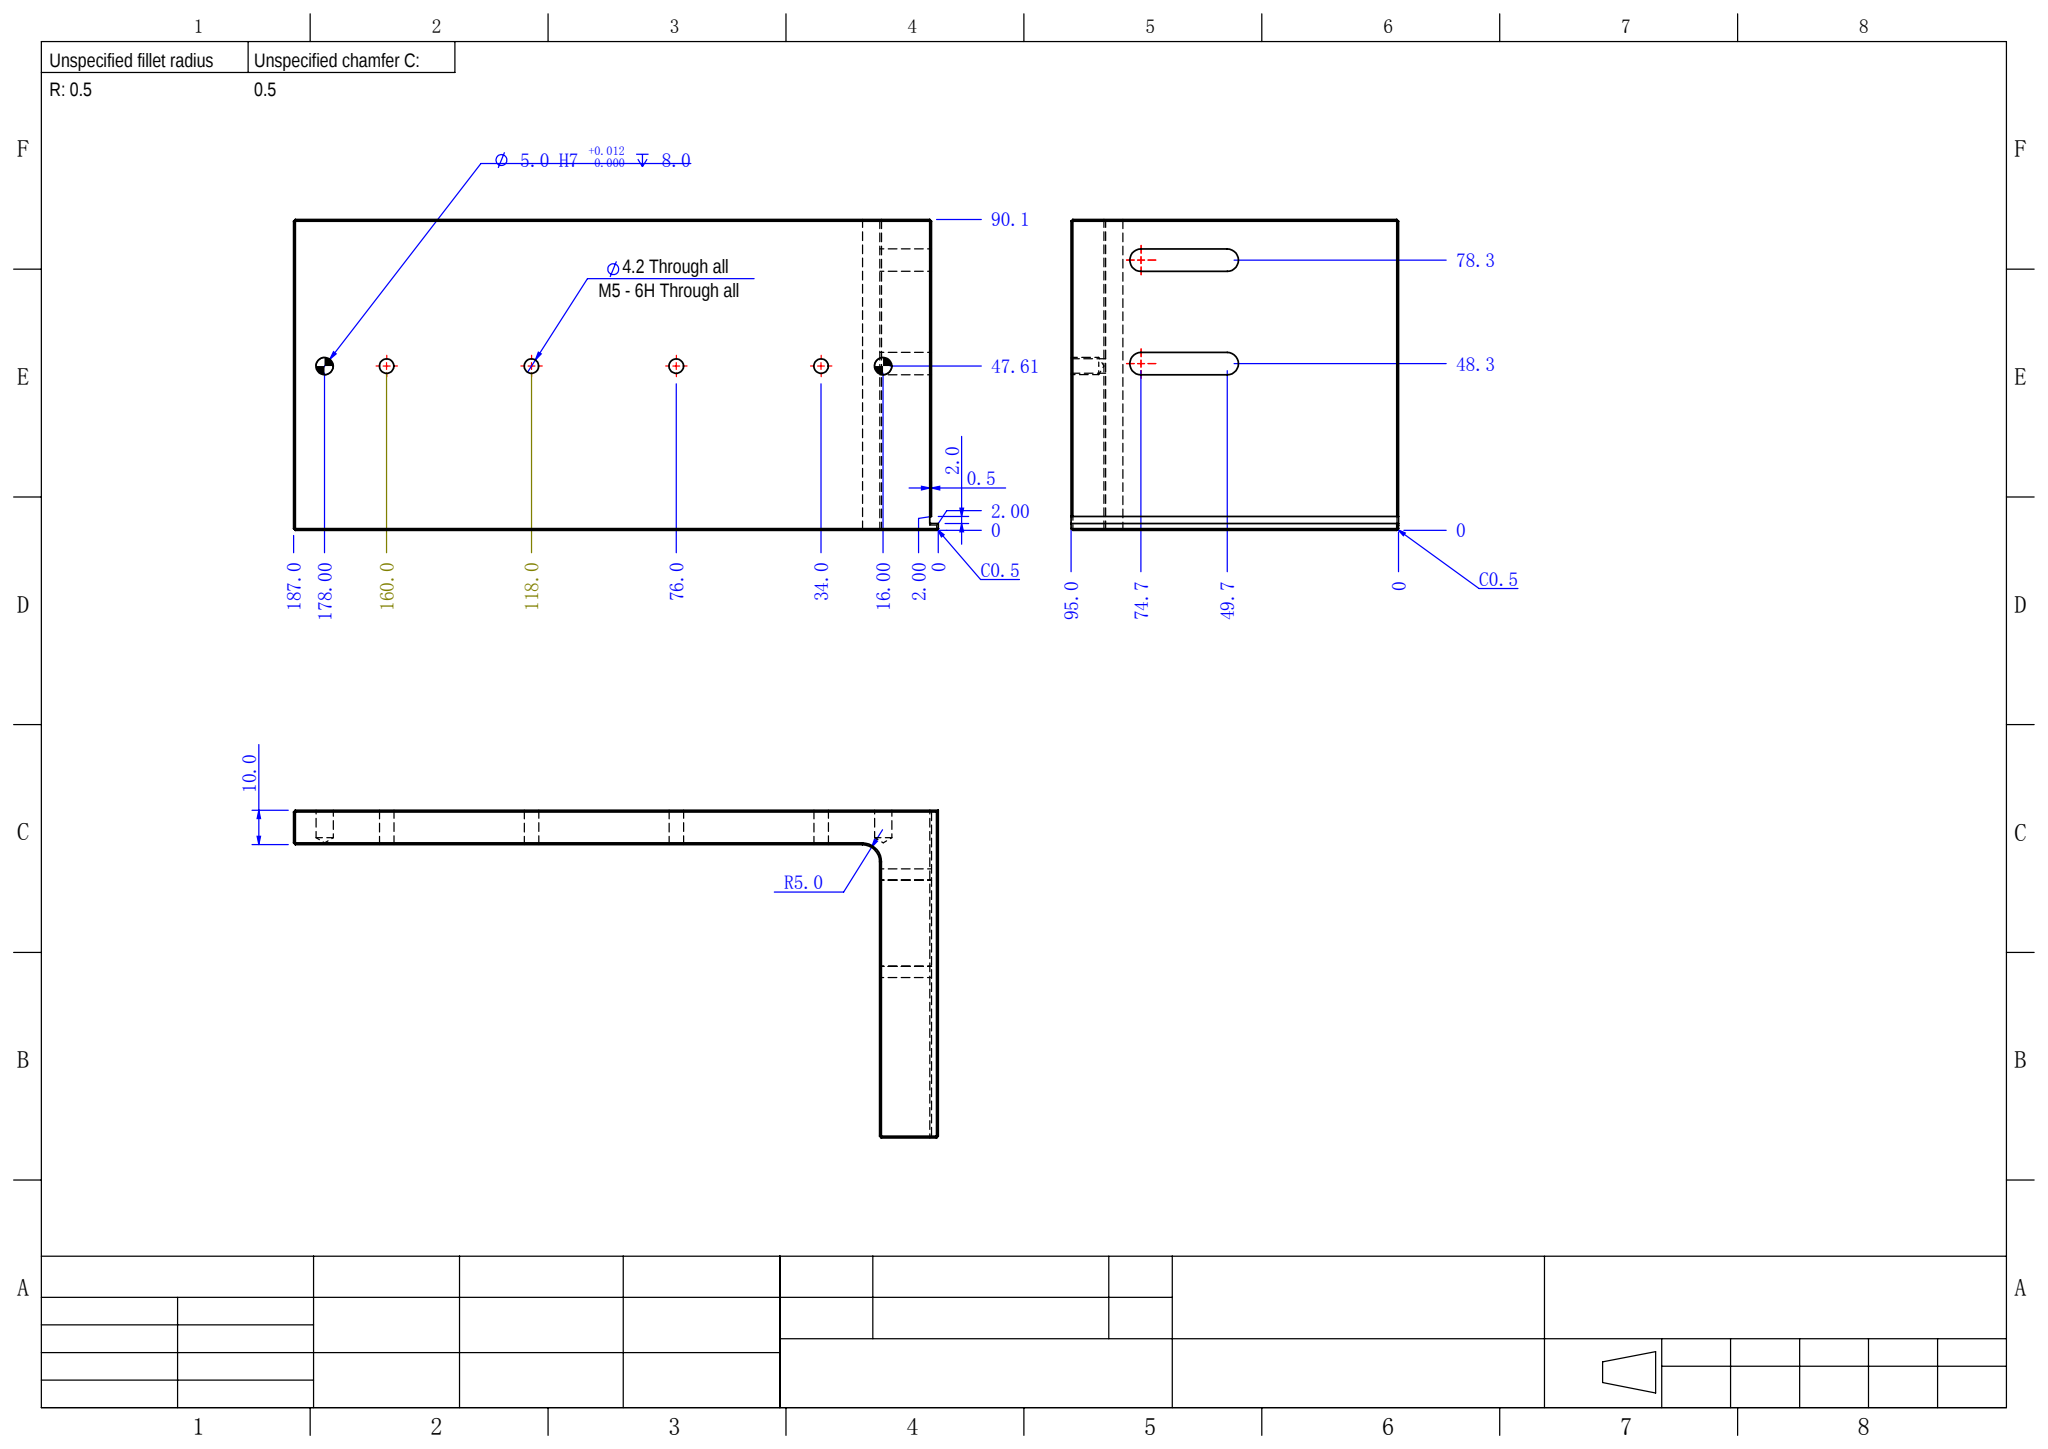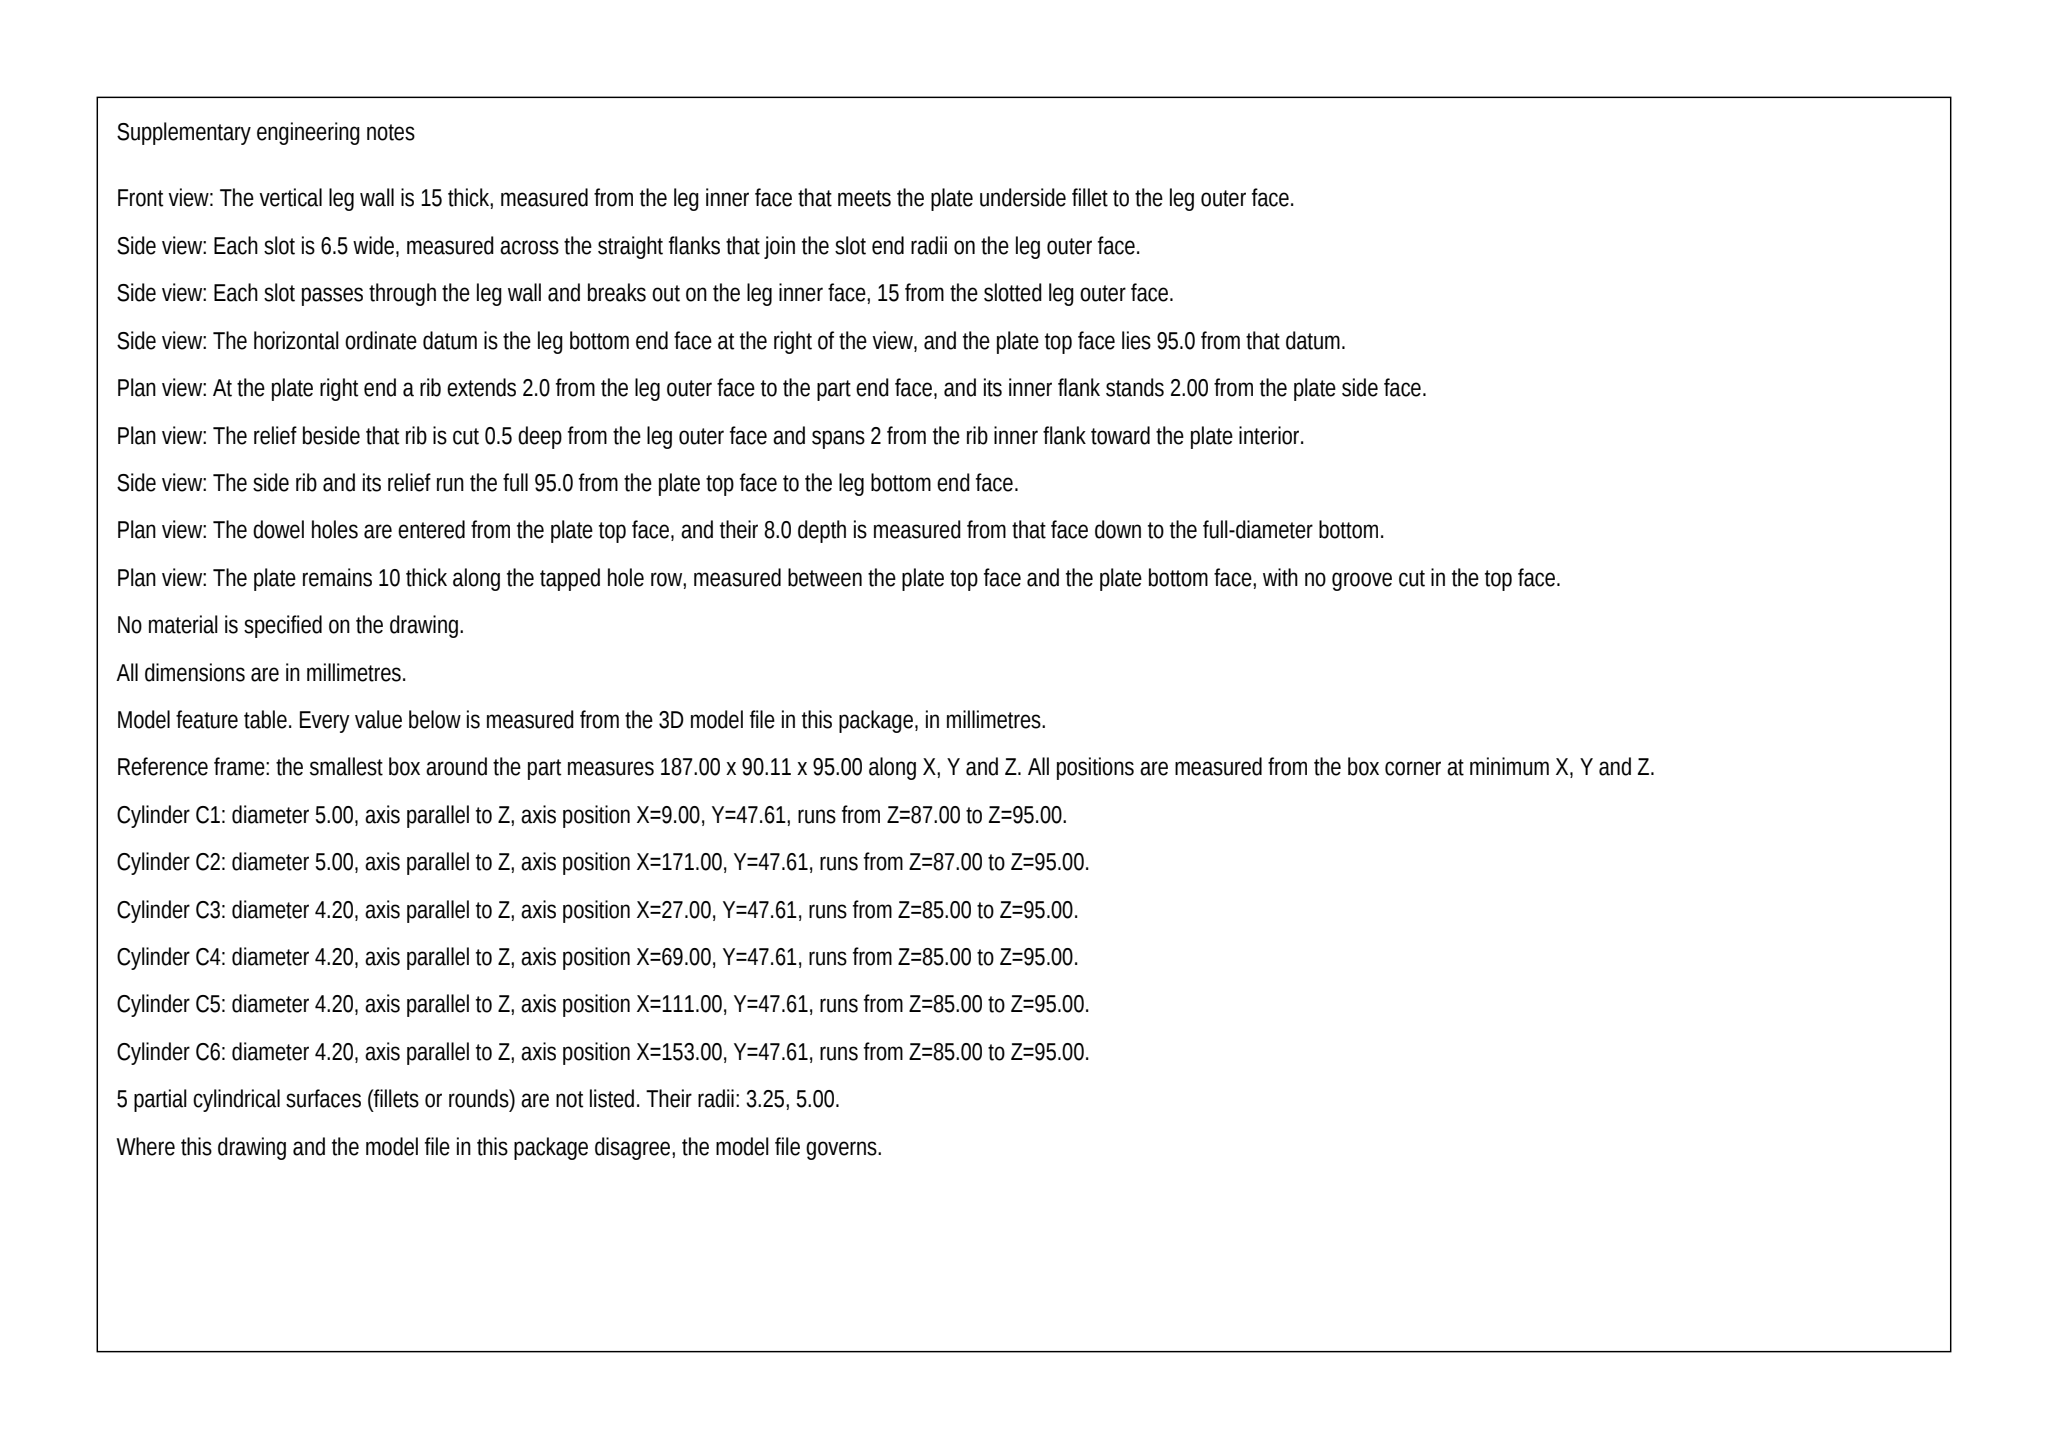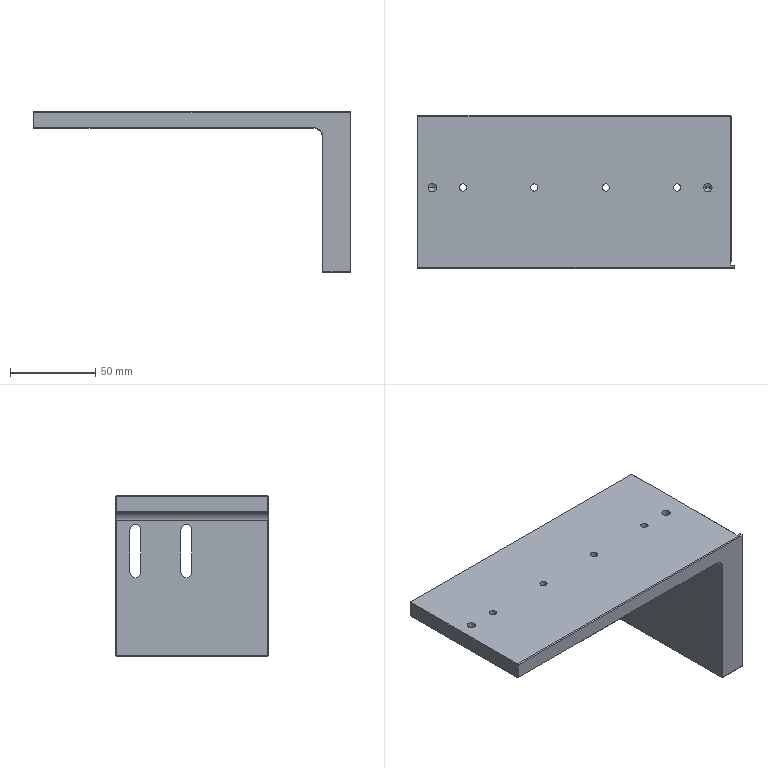Part | SolidWorks | mm | 1 solid | 70 faces | box 187 x 90.11 x 95 mm | volume 275409 mm3 | plane 45 | cylinder 19 | cone 6 | commonest cylinder face diameters 4.2 x8 6.5 x6 5 x4 10 x1
build123d program:
from build123d import *

# Parameters (mm, degrees)
SKETCH1_W                      = 180
SKETCH1_H                      = 65
BOSS_EXTRUDE1_DEPTH            = 10
M5_TAPPED_HOLE1_D              = 4.2
SIZE_MM_DOWEL_PIN_HOLE_1_D     = 5
SIZE_MM_DOWEL_PIN_HOLE_1_DEPTH = 8
SIZE_MM_DOWEL_PIN_HOLE_1_TIP   = 1.502
MOVE_FACE1_BY                  = 10
MOVE_FACE2_BY                  = 15.11
MOVE_FACE3_BY                  = 5
SKETCH6_W                      = 15
SKETCH6_H                      = 90.11
BOSS_EXTRUDE2_DEPTH            = 85
SKETCH8_W                      = 95
SKETCH8_H                      = 2
BOSS_EXTRUDE3_DEPTH            = 2
CUT_EXTRUDE1_DEPTH             = 205.328
CUT_EXTRUDE1_DEPTH_BACK        = 205.328
FILLET1_R                      = 5
CHAMFER1_SIZE                  = 0.5
SKETCH10_W                     = 95
SKETCH10_H                     = 2
CUT_EXTRUDE2_DEPTH             = 0.5


with BuildPart() as part:
    # Sketch1 → Boss-Extrude1 (new body)
    with BuildSketch(Plane.XY):
        with Locations((90, 32.5)):
            Rectangle(SKETCH1_W, SKETCH1_H)
    extrude(amount=BOSS_EXTRUDE1_DEPTH)

    # M5 Tapped Hole1 (through all)
    with Locations(Plane.XY.offset(10)):
        with Locations((69, 32.5), (27, 32.5), (111, 32.5), (153, 32.5)):
            Hole(M5_TAPPED_HOLE1_D / 2)

    # Size mm Dowel Pin Hole 1
    with Locations(Plane.XY.offset(10)):
        with Locations((9, 32.5), (171, 32.5)):
            Hole(SIZE_MM_DOWEL_PIN_HOLE_1_D / 2, depth=SIZE_MM_DOWEL_PIN_HOLE_1_DEPTH)
            with Locations((0, 0, -(SIZE_MM_DOWEL_PIN_HOLE_1_DEPTH + SIZE_MM_DOWEL_PIN_HOLE_1_TIP / 2))):  # 118° drill point
                Cone(0, SIZE_MM_DOWEL_PIN_HOLE_1_D / 2, SIZE_MM_DOWEL_PIN_HOLE_1_TIP, mode=Mode.SUBTRACT)

    # Move Face1: a face moved outward by 10.0
    extrude(part.faces().sort_by_distance((90, 65, 5))[0], amount=MOVE_FACE1_BY, dir=(0, 1, 0))

    # Move Face2: a face moved outward by 15.11
    extrude(part.faces().sort_by_distance((90, 0, 5))[0], amount=MOVE_FACE2_BY, dir=(0, -1, 0))

    # Move Face3: a face moved outward by 5.0
    extrude(part.faces().sort_by_distance((180, 29.945, 5))[0], amount=MOVE_FACE3_BY, dir=(1, 0, 0))

    # Sketch6 → Boss-Extrude2 (add)
    with BuildSketch(Plane(origin=(0, 0, 0), x_dir=(-1, 0, 0), z_dir=(0, 0, -1))):
        with Locations((-177.5, 29.945)):
            Rectangle(SKETCH6_W, SKETCH6_H)
    extrude(amount=BOSS_EXTRUDE2_DEPTH)

    # Sketch8 → Boss-Extrude3 (add)
    with BuildSketch(Plane(origin=(185, 0, 0), x_dir=(0, 0, -1), z_dir=(1, 0, 0))):
        with Locations((37.5, -14.11)):
            Rectangle(SKETCH8_W, SKETCH8_H)
    extrude(amount=BOSS_EXTRUDE3_DEPTH)

    # Sketch9 → Cut-Extrude1 (cut, two sides: drawn at the far end of the back side and taken through both)
    with BuildSketch(Plane.ZY.offset(-170).offset(-CUT_EXTRUDE1_DEPTH_BACK)):
        with BuildLine():
            Line((-10.29, 59.951), (-35.29, 59.951))
            ThreePointArc((-35.29, 59.951), (-38.54, 63.201), (-35.29, 66.451))
            Line((-35.29, 66.451), (-10.29, 66.451))
            ThreePointArc((-10.29, 66.451), (-7.04, 63.201), (-10.29, 59.951))
        make_face()
        with BuildLine():
            Line((-10.29, 29.951), (-35.29, 29.951))
            ThreePointArc((-35.29, 29.951), (-38.54, 33.201), (-35.29, 36.451))
            Line((-35.29, 36.451), (-10.29, 36.451))
            ThreePointArc((-10.29, 36.451), (-7.04, 33.201), (-10.29, 29.951))
        make_face()
    extrude(amount=CUT_EXTRUDE1_DEPTH + CUT_EXTRUDE1_DEPTH_BACK, mode=Mode.SUBTRACT)

    # Fillet1
    fillet1_edges = [part.edges().sort_by_distance(p)[0] for p in [
        (170, 29.945, 0),
    ]]
    fillet(fillet1_edges, radius=FILLET1_R)

    # Chamfer1
    chamfer1_edges = [part.edges().sort_by_distance(p)[0] for p in [
        (82.5, 75, 0),
        (168.536, 75, -1.464),
        (168.536, -15.11, -1.464),
        (92.5, 75, 10),
        (0, 29.945, 10),
        (170, -15.11, -45),
        (170, 75, -45),
        (185, 30.945, -85),
        (178.5, -15.11, -85),
        (170, 29.945, -85),
        (177.5, 75, -85),
        (82.5, -15.11, 0),
        (0, 29.945, 0),
        (185, 30.945, 10),
        (186, -13.11, -85),
        (187, -14.11, -85),
        (187, -15.11, -37.5),
        (0, 75, 5),
        (185, 75, -37.5),
        (0, -15.11, 5),
        (93.5, -15.11, 10),
    ]]
    chamfer(chamfer1_edges, length=CHAMFER1_SIZE)

    # Sketch10 → Cut-Extrude2 (cut)
    with BuildSketch(Plane(origin=(185, 0, 0), x_dir=(0, 0, -1), z_dir=(1, 0, 0))):
        with Locations((37.5, -12.11)):
            Rectangle(SKETCH10_W, SKETCH10_H)
    extrude(amount=-CUT_EXTRUDE2_DEPTH, mode=Mode.SUBTRACT)


solid = part.part